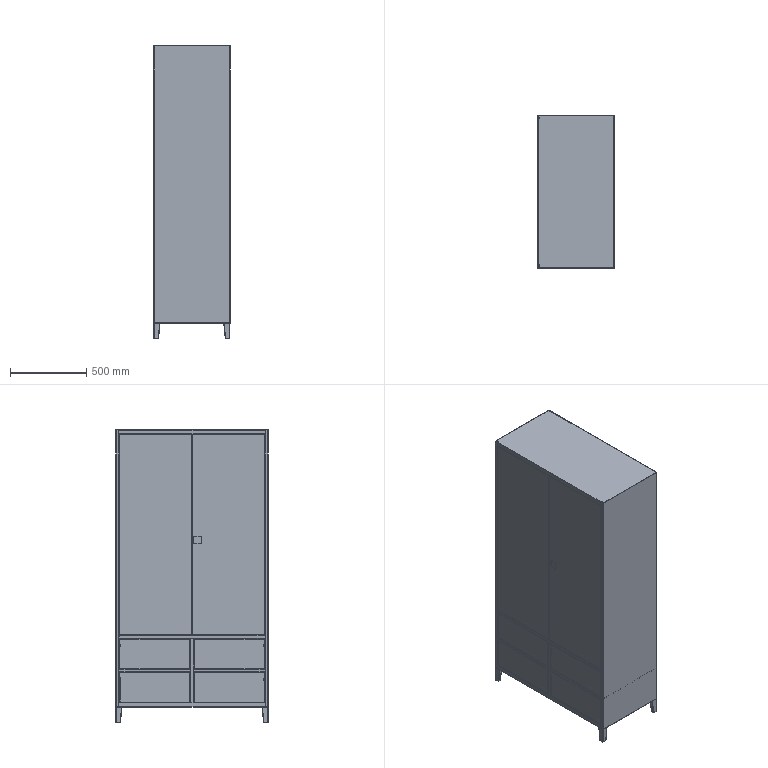Assembly | SolidWorks | mm | 23 component files | 23 solids | 959 faces | box 500 x 1000 x 1923 mm | volume 14431281 mm3 | plane 671 | cylinder 208 | spline 80 | commonest cylinder face diameters 2 x47 3 x46 5.4 x26 5 x22 6 x20 3.1 x12 0.1 x12 4.473 x9
Bill of materials:
BackPlate | 1 |  | Flat rectangular planar element with no visible thickness; looks like a single rectangular surface or a very thin sheet.
BottomPlate | 1 |  | Thin rectangular flat sheet with a short upturned flange along one long edge, ending in a small inward-bent return lip.
Drawer_Rib | 1 |  | Straight hollow square tube with rounded outer corners and uniform wall thickness, open at both ends.
Drawer | 4 |  | Open-top rectangular thin-walled tray/box: a flat bottom with four vertical side walls, one of which extends higher and ends in a small outward-turned lip.
DrawerStiffenerHorizontal | 2 |  | Straight hollow square tube with rounded outer corners, open at both ends; similar section to other square tubes but with a relatively thicker-looking wall.
DrawerStiffenerInner | 1 |  | Straight hollow rectangular tube (about 2:1 section) with rounded outer corners and thin uniform wall, open at both ends.
LeftDoor | 1 |  | Thin flat rectangular plate or panel with small edge rounding and no visible holes.
PartitionLeft | 1 |  | Near-square thin sheet panel with shallow down-turned edge flanges on at least two edges, and two rectangular notches cut into one edge.
PartitionRight | 1 |  | Near-square thin flat plate with two rectangular notches along one edge; edges appear slightly thickened or flanged.
RightDoor | 1 |  | Thin flat rectangular plate with one small square/rectangular through-cutout near one long edge, about mid-height.
Seat | 4 |  | Thin-walled, open-seam, roughly square hollow profile with rounded corners and an inward-stepped re-entrant corner channel along its length; side views suggest the profile tapers or is cut at an angle along one face.
Shelf | 1 |  | Thin rectangular flat sheet with a formed edge along one long side: a stepped offset plus a folded hollow rectangular hem/channel.
SidePlate | 2 |  | Thin, elongated rectangular sheet-like panel with short bent flanges along its two long edges; one edge flange ends in a small inward return (hook-like hem).
Stiffener | 1 |  | Straight, long hollow square tube with rounded outer corners and a uniform wall; both ends are cut square.
TopPlate | 1 |  | Flat rectangular sheet panel with shallow downturned flanges along its two long edges; one flange has a stepped, offset hook-like profile. It looks like a shallow tray or cover in shape.
Mates:
1. coincident | SidePlate-1 face at (-1.5, -254, 781.5) dir (-1, 0, 0) | TopPlate-2 face at (-1.5, 246, 1693) dir (-1, 0, 0)
2. coincident | SidePlate-1 face at (498.5, -252.5, 1691.5) dir (0, 0, 1) | TopPlate-2 face at (248.5, 246, 1691.5) dir (0, 0, -1)
3. coincident | SidePlate-1 face at (248.5, -234, 781.5) dir (0, 1, 0) | TopPlate-2 face at (-1.5, -234, 1691.5) dir (0, -1, 0)
4. coincident | TopPlate-2 face at (248.5, 246, 1691.5) dir (0, 0, -1) | SidePlate-2 face at (498.5, 744.5, 1691.5) dir (0, 0, 1)
5. coincident | TopPlate-2 face at (498.5, 746, 1691.5) dir (0, 1, 0) | SidePlate-2 face at (248.5, 746, 781.5) dir (0, 1, 0)
6. coincident | TopPlate-2 face at (498.5, 246, 1693) dir (1, 0, 0) | SidePlate-2 face at (498.5, 746, 781.5) dir (1, 0, 0)
7. coincident | SidePlate-1 face at (498.5, -252.5, -128.5) dir (0, 0, -1) | BottomPlate-2 face at (248.5, 246, -128.5) dir (0, 0, 1)
8. coincident | SidePlate-1 face at (-1.5, -254, 781.5) dir (-1, 0, 0) | BottomPlate-2 face at (-1.5, 246, -130) dir (-1, 0, 0)
9. coincident | SidePlate-1 face at (248.5, -234, 781.5) dir (0, 1, 0) | BottomPlate-2 face at (18.5, -234, -100) dir (0, -1, 0)
10. distance | Shelf-1 face at (-1.5, -234, 320) dir (0, 0, -1) | BottomPlate-2 face at (248.5, 246, -130) dir (0, 0, -1)
11. coincident | SidePlate-1 face at (248.5, -234, 781.5) dir (0, 1, 0) | Shelf-1 face at (13.5, -234, 343) dir (0, -1, 0)
12. coincident | SidePlate-1 face at (-1.5, -254, 781.5) dir (-1, 0, 0) | Shelf-1 face at (-1.5, -234, 343) dir (-1, 0, 0)
13. coincident | Shelf-1 face at (-1.5, -234, 320) dir (0, 0, -1) | Drawer_Rib-1 face at (-0.5, 237, 320) dir (0, 0, 1)
14. coincident | Shelf-1 face at (-1.5, -234, 343) dir (-1, 0, 0) | Drawer_Rib-1 face at (-1.5, 237, -100) dir (-1, 0, 0)
15. distance | Drawer_Rib-1 face at (17.5, 256, -100) dir (0, 1, 0) | SidePlate-2 face at (248.5, 726, 781.5) dir (0, -1, 0)
16. coincident | SidePlate-2 face at (-1.5, 746, 781.5) dir (-1, 0, 0) | DrawerStiffenerHorizontal-1 face at (-1.5, 726, 119) dir (-1, 0, 0)
17. coincident | SidePlate-2 face at (248.5, 726, 781.5) dir (0, -1, 0) | DrawerStiffenerHorizontal-1 face at (-0.5, 726, 119) dir (0, 1, 0)
18. distance | DrawerStiffenerHorizontal-1 face at (-0.5, 726, 100) dir (0, 0, -1) | BottomPlate-2 face at (248.5, 246, -130) dir (0, 0, -1)
19. coincident | Drawer_Rib-1 face at (-1.5, 237, -100) dir (-1, 0, 0) | DrawerStiffenerHorizontal-2 face at (-1.5, -234, 119) dir (-1, 0, 0)
20. coincident | SidePlate-1 face at (248.5, -234, 781.5) dir (0, 1, 0) | DrawerStiffenerHorizontal-2 face at (17.5, -234, 119) dir (0, -1, 0)
21. distance | DrawerStiffenerHorizontal-2 face at (17.5, -234, 100) dir (0, 0, -1) | BottomPlate-2 face at (248.5, 246, -130) dir (0, 0, -1)
22. coincident | SidePlate-2 face at (497, 746, 781.5) dir (-1, 0, 0) | BackPlate-3 face at (497, 246, 781.5) dir (1, 0, 0)
23. coincident | TopPlate-2 face at (248.5, 246, 1691.5) dir (0, 0, -1) | BackPlate-3 face at (497, -252.5, 1691.5) dir (0, 0, 1)
24. coincident | SidePlate-1 face at (248.5, -252.5, 781.5) dir (0, 1, 0) | BackPlate-3 face at (497, -252.5, -128.5) dir (0, -1, 0)
25. coincident | BottomPlate-2 face at (248.5, 246, -128.5) dir (0, 0, 1) | DrawerStiffenerInner-1 face at (19.5, 237, -128.5) dir (0, 0, -1)
26. coincident | Drawer_Rib-1 face at (17.5, 236, -100) dir (0, -1, 0) | DrawerStiffenerInner-1 face at (57.5, 236, -128.5) dir (0, -1, 0)
27. distance | DrawerStiffenerInner-1 face at (18.5, 237, -128.5) dir (-1, 0, 0) | Drawer_Rib-1 face at (-1.5, 237, -100) dir (-1, 0, 0)
28. coincident | Shelf-1 face at (56.844, -234, 351.8) dir (0, 0, -1) | Stiffener-1 face at (217.5, 237, 351.8) dir (0, 0, 1)
29. coincident | DrawerStiffenerInner-1 face at (57.5, 256, -128.5) dir (0, 1, 0) | Stiffener-1 face at (217.5, 256, 351.8) dir (0, 1, 0)
30. distance | Stiffener-1 face at (198.5, 237, 351.8) dir (-1, 0, 0) | Drawer_Rib-1 face at (-1.5, 237, -100) dir (-1, 0, 0)
31. coincident | DrawerStiffenerHorizontal-1 face at (-0.5, 726, 120) dir (0, 0, 1) | PartitionLeft-1 face at (257.9, 492.483, 120) dir (0, 0, 1)
32. distance | PartitionLeft-1 face at (18.5, 492.483, 120) dir (-1, 0, 0) | DrawerStiffenerHorizontal-1 face at (-1.5, 726, 119) dir (-1, 0, 0)
33. coincident | DrawerStiffenerInner-1 face at (57.5, 256, -128.5) dir (0, 1, 0) | PartitionLeft-1 face at (18.5, 256, 118.8) dir (0, -1, 0)
34. coincident | DrawerStiffenerHorizontal-2 face at (17.5, -234, 120) dir (0, 0, 1) | PartitionRight-1 face at (257.9, -0.483, 120) dir (0, 0, 1)
35. coincident | DrawerStiffenerInner-1 face at (57.5, 236, -128.5) dir (0, -1, 0) | PartitionRight-1 face at (18.5, 236, 120) dir (0, 1, 0)
36. distance | PartitionRight-1 face at (18.5, -0.483, 118.8) dir (-1, 0, 0) | DrawerStiffenerHorizontal-2 face at (-1.5, -234, 119) dir (-1, 0, 0)
37. coincident | BottomPlate-2 face at (248.5, 246, -130) dir (0, 0, -1) | Seat-1 face at (494.3, 743.3, -130) dir (0, 0, 1)
38. coincident | BackPlate-3 face at (497, 246, 781.5) dir (1, 0, 0) | Seat-1 face at (497, 726, -180) dir (1, 0, 0)
39. coincident | SidePlate-2 face at (248.5, 746, 781.5) dir (0, 1, 0) | Seat-1 face at (495.8, 746, -180) dir (0, 1, 0)
40. coincident | BottomPlate-2 face at (248.5, 246, -130) dir (0, 0, -1) | Seat-4 face at (1.2, -251.3, -130) dir (0, 0, 1)
41. coincident | SidePlate-1 face at (-1.5, -254, 781.5) dir (-1, 0, 0) | Seat-4 face at (-1.5, -234, -180) dir (-1, 0, 0)
42. coincident | SidePlate-1 face at (248.5, -254, 781.5) dir (0, -1, 0) | Seat-4 face at (-0.3, -254, -180) dir (0, -1, 0)
43. coincident | BottomPlate-2 face at (248.5, 246, -130) dir (0, 0, -1) | Seat-5 face at (1.2, 743.3, -130) dir (0, 0, 1)
44. coincident | BottomPlate-2 face at (-1.5, 246, -130) dir (-1, 0, 0) | Seat-5 face at (-1.5, 744.8, -180) dir (-1, 0, 0)
45. coincident | SidePlate-2 face at (248.5, 746, 781.5) dir (0, 1, 0) | Seat-5 face at (18.5, 746, -180) dir (0, 1, 0)
46. coincident | BottomPlate-2 face at (248.5, 246, -130) dir (0, 0, -1) | Seat-6 face at (494.3, -251.3, -130) dir (0, 0, 1)
47. coincident | BackPlate-3 face at (497, 246, 781.5) dir (1, 0, 0) | Seat-6 face at (497, -252.8, -180) dir (1, 0, 0)
48. coincident | SidePlate-1 face at (248.5, -254, 781.5) dir (0, -1, 0) | Seat-6 face at (477, -254, -180) dir (0, -1, 0)
49. coincident | Drawer_Rib-1 face at (-1.5, 237, -100) dir (-1, 0, 0) | Drawer-1 face at (-1.5, 1, 220) dir (-1, 0, 0)
50. coincident | DrawerStiffenerHorizontal-1 face at (-0.5, 726, 120) dir (0, 0, 1) | Drawer-1 face at (0, 1, 120) dir (0, 0, -1)
51. distance | Drawer-1 face at (0, 231, 220) dir (0, 1, 0) | SidePlate-2 face at (248.5, 726, 781.5) dir (0, -1, 0)
52. coincident | DrawerStiffenerHorizontal-2 face at (-1.5, -234, 119) dir (-1, 0, 0) | Drawer-3 face at (-1.5, 0, 0) dir (-1, 0, 0)
53. coincident | BottomPlate-2 face at (248.5, 246, -100) dir (0, 0, 1) | Drawer-3 face at (0, 0, -100) dir (0, 0, -1)
54. distance | SidePlate-1 face at (248.5, -234, 781.5) dir (0, 1, 0) | Drawer-3 face at (0, -230, 0) dir (0, -1, 0)
55. coincident | SidePlate-2 face at (-1.5, 746, 781.5) dir (-1, 0, 0) | LeftDoor-1 face at (-1.5, 486.5, 1003) dir (-1, 0, 0)
56. coincident | Shelf-1 face at (13.5, -234, 343) dir (0, 0, 1) | LeftDoor-1 face at (0, 486.5, 343) dir (0, 0, -1)
57. coincident | SidePlate-2 face at (248.5, 726, 781.5) dir (0, -1, 0) | LeftDoor-1 face at (0, 726, 1003) dir (0, 1, 0)
58. coincident | SidePlate-1 face at (-1.5, -254, 781.5) dir (-1, 0, 0) | RightDoor-1 face at (-1.5, 5.5, 1003) dir (-1, 0, 0)
59. coincident | Shelf-1 face at (13.5, -234, 343) dir (0, 0, 1) | RightDoor-1 face at (0, 5.5, 343) dir (0, 0, -1)
60. coincident | SidePlate-1 face at (248.5, -234, 781.5) dir (0, 1, 0) | RightDoor-1 face at (0, -234, 1003) dir (0, -1, 0)